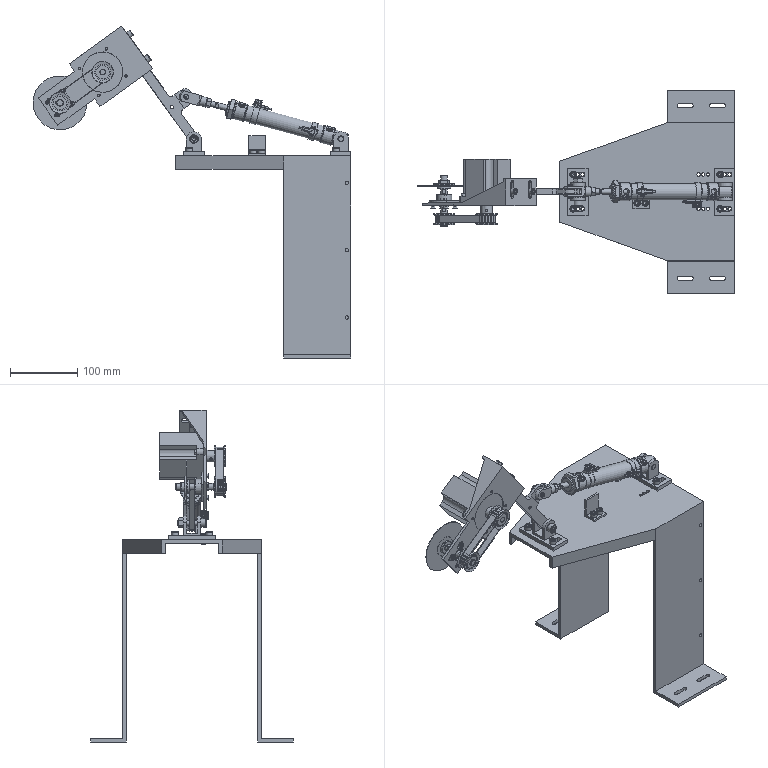Assembly | NX | mm | 40 component files | 66 solids | 1547 faces | box 471.68 x 300 x 492.56 mm | volume 1051873 mm3 | plane 738 | cylinder 525 | cone 205 | torus 53 | sphere 24 | spline 2 | commonest cylinder face diameters 6.55 x68 0.5 x67 1.1 x66 24.5 x35 20.96 x34 5 x26 10 x21 3.838 x16
Bill of materials:
unnamed part 1 | 1 |  | Long slender cylindrical rod. One end has a short smaller-diameter stub, a hexagonal collar or nut, a short cylindrical section and a narrow groove before the main shaft. The other end is plain and flat.
unnamed part 2 | 2 |  | Clevis-style bracket: a flat rectangular base plate with two parallel upright lugs. Each lug has a rounded top and one through-hole, and the holes line up. The base has two elongated slots, one at each end.
unnamed part 3 | 1 |  | Toothed pulley with a flange on each side. The flanges have angled inner faces. The center bore has a keyway, and there is no hub extension. A small radial hole or feature shows in one tooth groove.
unnamed part 4 | 1 |  | Toothed pulley with flanges on both sides, a plain round bore and a cylindrical hub on one side. The hub has one radial hole.
unnamed part 5 | 1 |  | Cylindrical rod or pin with a hexagonal head at one end and a shorter reduced-diameter end at the other. The reduced end has a cross-hole and a flat. Two collar-like bands sit on the shaft, each with a cross-hole and a small hex-head fastener beside it. The end of the hex head shows a recess or hole.
unnamed part 6 | 1 |  | Flanged bushing or washer: a thin round flange with chamfered edges and a short cylindrical boss on one face, with a through-bore. A counterbore or step is visible in the bore on the flange side.
unnamed part 7 | 1 |  | Flanged housing: a plate flange that is mostly round with two parallel flat sides. It has four small through-holes and a large central bore. A cylindrical boss projects from one face, and the bore has an internal step or shoulder.
unnamed part 8 | 1 |  | L-shaped angle bracket made of two flat rectangular legs at a right angle. The horizontal leg has two round through-holes, and the vertical leg has no visible features.
GB-T70.1-2000,M6x10 | 6 |  | Hexagon Socket Head Cap Screw, GB-T 70.1-2000,M6x10
GB-T70.1-2000,M8x35 | 1 |  | Hexagon Socket Head Cap Screw, GB-T 70.1-2000,M8x35
unnamed part 9 | 1 |  | Stepped cylindrical shaft or stud with an integral two-step collar near one end. The longer side of the shaft has several shallow circumferential steps or grooves with small notches, and both ends are chamfered.
unnamed part 10 | 2 |  | Circular band clamp: a thin cylindrical ring with a rectangular block-type tightening housing on the outside. A cylindrical pin projects tangentially from the housing, and a domed, rivet-like head sits on the housing.
unnamed part 11 | 1 |  | Square-body motor-like unit: a square flange with rounded corners and four through-holes, and a square body with long recessed grooves on its corners. A short round boss and a single cylindrical shaft project from the flange face.
unnamed part 12 | 1 |  | Flat thin bar or link with rounded ends. A lobed tab sticks out sideways near the middle and has a larger hole. The bar has round holes near each end and along its length, plus a small hole near the tab.
GB-T70.1-2000,M4x12 | 4 |  | Hexagon Socket Head Cap Screw, GB-T 70.1-2000,M4x12
unnamed part 13 | 1 |  | Very thin flat annular disc (washer-like ring) with a single concentric circular through-hole.
unnamed part 14 | 2 |  | Ball-bearing-like ring assembly: concentric outer and inner rings with a circle of spherical balls between them; no cage or shields visible.
unnamed part 15 | 1 |  | Clevis/fork-type body: a block with two parallel prongs separated by a rectangular slot, a cylindrical shank with an axial bore at one end, and a headed cylindrical pin passing crosswise through both prongs.
GB-T70.1-2000,M4x6 | 4 |  | Hexagon Socket Head Cap Screw, GB-T 70.1-2000,M4x6
GB-T6170_F-2000,M8x1.25 | 1 |  | Hexagonal nut-like body: hex prism with a central cylindrical through-bore and chamfered corners on both end faces.
unnamed part 16 | 1 |  | Hat-shaped (U-channel) sheet-metal bracket: a top plate with a tapered extension, two vertical legs, and outward foot flanges with slots.
unnamed part 17 | 1 |  | L-shaped plate bracket: a stepped main plate with a large circular opening and a smaller circular opening, a perpendicular flange with two long slots, and a triangular gusset.
GB-T70.1-2000,M6x16 | 2 |  | Hexagon Socket Head Cap Screw, GB-T 70.1-2000,M6x16
unnamed part 18 | 1 |  | Thin-walled obround (stadium-shaped) closed band/ring that is open at both ends, with uniform wall thickness and a short height.
GB-T119.1-2000,8x26 | 1 |  | Parallel Pin, GB-T 119.1-2000,8x26
Mates:
1. concentric | Bearing_Sleeve 1 edge | Motor_Mounting_Plate 1 edge
2. concentric | Bearing_61800 2 edge | Bearing_Sleeve 1 edge
3. concentric | Bearing_61800 1 edge | Bearing_Sleeve 1 edge
4. concentric | Mounting_Shaft 1 edge | Bearing_61800 2 edge
5. concentric | Synchronous_Pulley_1 1 edge | Mounting_Shaft 1 edge
6. concentric | Blade 1 edge | Mounting_Shaft 1 edge
7. concentric | Blade 1 edge | Lock_Nut 1 edge
8. touch align | Motor 1 face | Motor_Mounting_Plate 1 face
9. concentric | Motor 1 edge | Motor_Mounting_Plate 1 edge
10. touch align | Synchronous_Pulley_2 1 face | Motor 1 face
11. touch align | Synchronous_Pulley_2 1 face | Synchronous_Pulley_1 1 face
12. concentric | Belt 1 edge | Synchronous_Pulley_1 1 edge
13. touch align | Belt 1 face | Synchronous_Pulley_2 1 face
14. touch align | Connecting_Rod 1 face | Motor_Mounting_Plate 1 face
15. touch align | Connecting_Rod 1 face | Motor_Mounting_Plate 1 face
16. distance | Connecting_Rod 1 face | Motor_Mounting_Plate 1 face
17. touch align | Fixed_Mount 2 face | Support_Plate 1 face
18. fix | Support_Plate 1 component
19. touch align | Fixed_Mount 2 face | Support_Plate 1 face
20. concentric | Mini_Cylinder 1 edge | Fixed_Mount 2 edge
21. concentric | Fixed_Mount 1 edge | Support_Plate 1 arc
22. touch align | Connecting_Rod 1 face | Fixed_Mount 1 face
23. center | Connecting_Rod 1 face | Connecting_Rod 1 face | Fixed_Mount 1 face | Fixed_Mount 1 face
24. concentric | F-MA20Y 1 edge | Mini_Cylinder 1 edge
25. parallel | Fixed_Mount 2 face | Support_Plate 1 face
26. touch align | F-MA20Y 1 face | Connecting_Rod 1 face
27. parallel | Bearing_Sleeve 1 face | Motor_Mounting_Plate 1 face
28. concentric | Nut_M8 1 edge | Fixed_Mount 1 edge
29. touch align | Screw_M6x16 2 face | Connecting_Rod 1 face
30. touch align | Screw_M6x16 1 face | Connecting_Rod 1 edge
31. touch align | Screw_M6x16 2 face | Motor_Mounting_Plate 1 face
32. touch align | Screw_M6x16 1 face | Motor_Mounting_Plate 1 face
33. concentric | Screw_M4x12 1 edge | Motor 1 edge
34. concentric | Screw_M4x12 3 edge | Motor 1 edge
35. concentric | Screw_M4x12 2 edge | Motor 1 edge
36. concentric | Screw_M4x12 4 edge | Motor 1 edge
37. touch align | Screw_M4x6 4 face | Bearing_Sleeve 1 face
38. touch align | Screw_M4x6 4 face | Motor_Mounting_Plate 1 face
39. bond | Bearing_Sleeve 1 component | assembly component
40. bond | Screw_M4x6 4 component | assembly component
41. bond | Screw_M4x6 3 component | assembly component
42. bond | Screw_M4x6 2 component | assembly component
43. bond | Screw_M4x6 1 component | assembly component
44. circular | assembly datumaxis | assembly cartesiancoordinatesystem | assembly cartesiancoordinatesystem | assembly cartesiancoordinatesystem | assembly cartesiancoordinatesystem
45. concentric | Spring_Fixing_Plate 1 edge | Support_Plate 1 arc
46. concentric | Screw_M6x10 2 edge | Spring_Fixing_Plate 1 edge
47. concentric | Screw_M6x10 1 edge | Spring_Fixing_Plate 1 edge